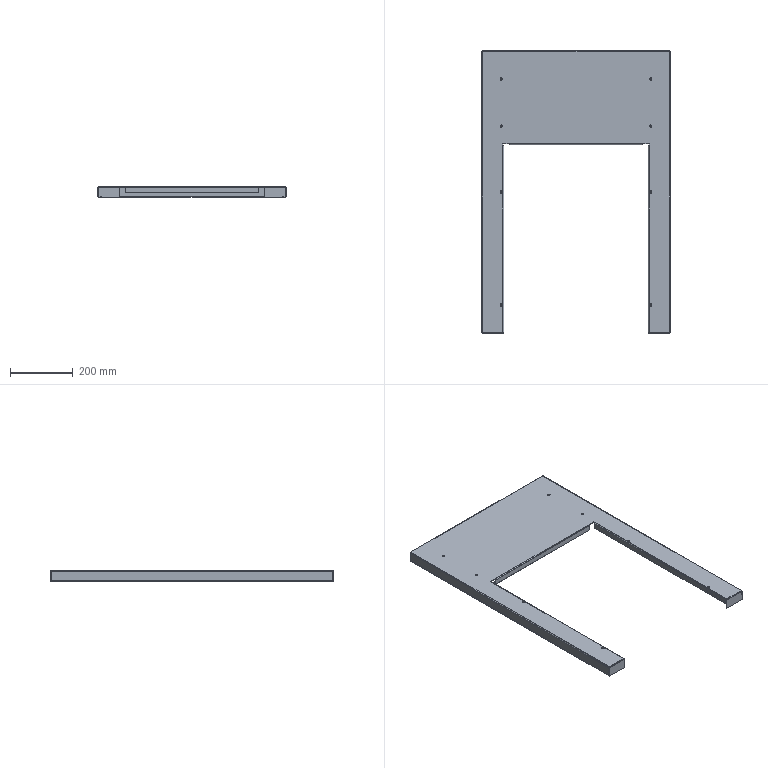Component | SolidWorks | UpperSeatAssembly-1_UpperSeat2-1 | 1 solid | 140 faces | volume 787077 mm3 | plane 70 | cylinder 58 | spline 12 | commonest cylinder face diameters 6.8 x20 7 x16 6 x11 2 x11